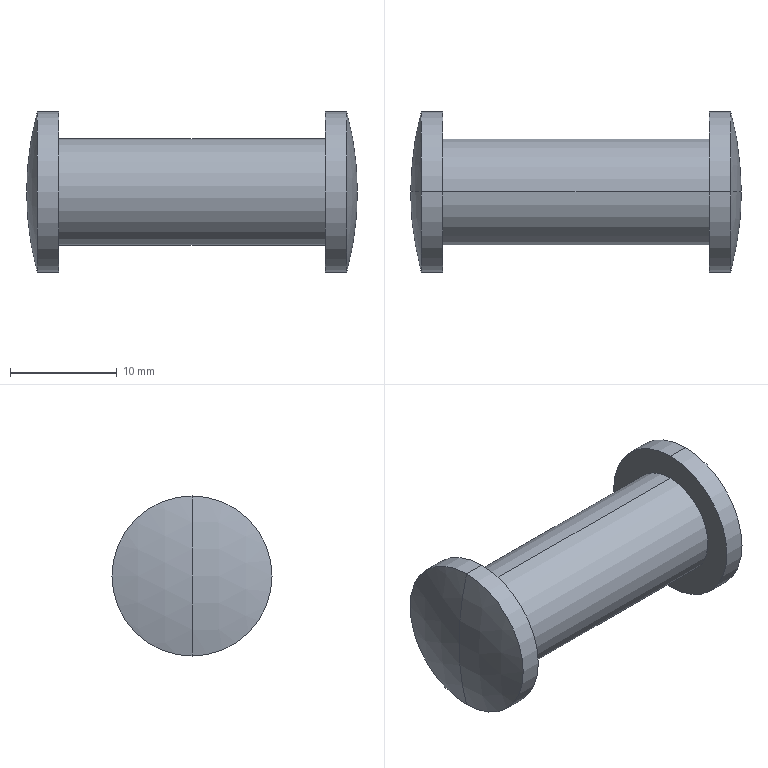Component | SolidWorks | 10x25DowelPin-1 | 1 solid | 12 faces | box 31 x 15 x 15 mm | volume 2848 mm3 | cylinder 6 | sphere 4 | plane 2 | commonest cylinder face diameters 15 x4 10 x2
build123d program:
from build123d import *

# Parameters (mm, degrees)
SKETCH1_R           = 5
BOSS_EXTRUDE1_DEPTH = 12.5
SKETCH2_R           = 7.5
BOSS_EXTRUDE2_DEPTH = 2
DOME1_FACE_RADIUS   = 7.5
DOME1_HEIGHT        = 1
DOME2_FACE_RADIUS   = 7.5
DOME2_HEIGHT        = 1


with BuildPart() as part:
    # Sketch1 → Boss-Extrude1 (new, symmetric)
    with BuildSketch(Plane.XY):
        Circle(SKETCH1_R)
    extrude(amount=BOSS_EXTRUDE1_DEPTH, both=True)

    # Sketch2 → Boss-Extrude2 (add)
    with BuildSketch(Plane.XY.offset(12.5)):
        Circle(SKETCH2_R)
    boss_extrude2 = extrude(amount=BOSS_EXTRUDE2_DEPTH)

    # Mirror1: Boss-Extrude2 across plane
    add(boss_extrude2.mirror(Plane.XY))

    # Dome1: a dome of height H over a round flat face of radius A is a cap of a sphere of radius (A * A + H * H) / (2 * H)
    dome1_r = (DOME1_FACE_RADIUS * DOME1_FACE_RADIUS + DOME1_HEIGHT * DOME1_HEIGHT) / (2 * DOME1_HEIGHT)
    dome1_base = Plane((0, 0, 14.5), z_dir=(0, 0, 1))
    with Locations(dome1_base.offset(DOME1_HEIGHT - dome1_r)):
        dome1_ball = Sphere(dome1_r, mode=Mode.PRIVATE)
    add(split(dome1_ball, bisect_by=dome1_base, keep=Keep.TOP, mode=Mode.PRIVATE))

    # Dome2: a dome of height H over a round flat face of radius A is a cap of a sphere of radius (A * A + H * H) / (2 * H)
    dome2_r = (DOME2_FACE_RADIUS * DOME2_FACE_RADIUS + DOME2_HEIGHT * DOME2_HEIGHT) / (2 * DOME2_HEIGHT)
    dome2_base = Plane((0, 0, -14.5), z_dir=(0, 0, -1))
    with Locations(dome2_base.offset(DOME2_HEIGHT - dome2_r)):
        dome2_ball = Sphere(dome2_r, mode=Mode.PRIVATE)
    add(split(dome2_ball, bisect_by=dome2_base, keep=Keep.TOP, mode=Mode.PRIVATE))


solid = part.part

# Placed as in the assembly
solid = solid.moved(Location((0, -60.308, -258.214), (0, 90, 0)))
STEP:
#1=COLOUR_RGB('',0.7922,0.8196,0.9333);
#2=FILL_AREA_STYLE_COLOUR('',#1);
#3=FILL_AREA_STYLE('',(#2));
#4=SURFACE_STYLE_FILL_AREA(#3);
#5=SURFACE_SIDE_STYLE('',(#4));
#6=SURFACE_STYLE_USAGE(.BOTH.,#5);
#7=PRESENTATION_STYLE_ASSIGNMENT((#6));
#8=CARTESIAN_POINT('',(0.6102,-2.374,-10.166));
#9=VERTEX_POINT('',#8);
#10=CARTESIAN_POINT('',(0.5709,-2.374,-9.871));
#11=VERTEX_POINT('',#10);
#12=CARTESIAN_POINT('',(-0.5167,-2.374,-10.166));
#13=DIRECTION('',(0.,-1.,0.));
#14=DIRECTION('',(0.,0.,-1.));
#15=AXIS2_PLACEMENT_3D('',#12,#13,#14);
#16=CIRCLE('',#15,1.127);
#17=EDGE_CURVE('',#9,#11,#16,.T.);
#18=ORIENTED_EDGE('',*,*,#17,.F.);
#19=CARTESIAN_POINT('',(0.5709,-2.374,-10.461));
#20=VERTEX_POINT('',#19);
#21=CARTESIAN_POINT('',(-0.5167,-2.374,-10.166));
#22=DIRECTION('',(0.,1.,0.));
#23=DIRECTION('',(0.,-0.,1.));
#24=AXIS2_PLACEMENT_3D('',#21,#22,#23);
#25=CIRCLE('',#24,1.127);
#26=EDGE_CURVE('',#9,#20,#25,.T.);
#27=ORIENTED_EDGE('',*,*,#26,.T.);
#28=CARTESIAN_POINT('',(0.5709,-2.374,-10.166));
#29=DIRECTION('',(-1.,0.,0.));
#30=DIRECTION('',(0.,0.,1.));
#31=AXIS2_PLACEMENT_3D('',#28,#29,#30);
#32=CIRCLE('',#31,0.2953);
#33=EDGE_CURVE('',#11,#20,#32,.T.);
#34=ORIENTED_EDGE('',*,*,#33,.F.);
#35=EDGE_LOOP('',(#18,#27,#34));
#36=FACE_OUTER_BOUND('',#35,.T.);
#37=CARTESIAN_POINT('',(-0.5167,-2.374,-10.166));
#38=DIRECTION('',(0.,1.,0.));
#39=DIRECTION('',(0.,0.,1.));
#40=AXIS2_PLACEMENT_3D('',#37,#38,#39);
#41=SPHERICAL_SURFACE('',#40,1.127);
#42=ADVANCED_FACE('',(#36),#41,.T.);
#43=ORIENTED_EDGE('',*,*,#33,.T.);
#44=CARTESIAN_POINT('',(0.4921,-2.374,-10.461));
#45=VERTEX_POINT('',#44);
#46=CARTESIAN_POINT('',(0.5709,-2.374,-10.461));
#47=DIRECTION('',(-1.,0.,0.));
#48=VECTOR('',#47,39.37);
#49=LINE('',#46,#48);
#50=EDGE_CURVE('',#20,#45,#49,.T.);
#51=ORIENTED_EDGE('',*,*,#50,.T.);
#52=CARTESIAN_POINT('',(0.4921,-2.374,-9.871));
#53=VERTEX_POINT('',#52);
#54=CARTESIAN_POINT('',(0.4921,-2.374,-10.166));
#55=DIRECTION('',(-1.,0.,0.));
#56=DIRECTION('',(0.,0.,1.));
#57=AXIS2_PLACEMENT_3D('',#54,#55,#56);
#58=CIRCLE('',#57,0.2953);
#59=EDGE_CURVE('',#53,#45,#58,.T.);
#60=ORIENTED_EDGE('',*,*,#59,.F.);
#61=CARTESIAN_POINT('',(0.5709,-2.374,-9.871));
#62=DIRECTION('',(-1.,0.,0.));
#63=VECTOR('',#62,39.37);
#64=LINE('',#61,#63);
#65=EDGE_CURVE('',#11,#53,#64,.T.);
#66=ORIENTED_EDGE('',*,*,#65,.F.);
#67=EDGE_LOOP('',(#43,#51,#60,#66));
#68=FACE_OUTER_BOUND('',#67,.T.);
#69=CARTESIAN_POINT('',(0.5709,-2.374,-10.166));
#70=DIRECTION('',(-1.,0.,0.));
#71=DIRECTION('',(0.,0.,1.));
#72=AXIS2_PLACEMENT_3D('',#69,#70,#71);
#73=CYLINDRICAL_SURFACE('',#72,0.2953);
#74=ADVANCED_FACE('',(#68),#73,.T.);
#75=CARTESIAN_POINT('',(-0.5709,-2.374,-9.871));
#76=VERTEX_POINT('',#75);
#77=CARTESIAN_POINT('',(-0.5709,-2.374,-10.461));
#78=VERTEX_POINT('',#77);
#79=CARTESIAN_POINT('',(-0.5709,-2.374,-10.166));
#80=DIRECTION('',(-1.,0.,0.));
#81=DIRECTION('',(0.,0.,1.));
#82=AXIS2_PLACEMENT_3D('',#79,#80,#81);
#83=CIRCLE('',#82,0.2953);
#84=EDGE_CURVE('',#76,#78,#83,.T.);
#85=ORIENTED_EDGE('',*,*,#84,.T.);
#86=CARTESIAN_POINT('',(-0.6102,-2.374,-10.166));
#87=VERTEX_POINT('',#86);
#88=CARTESIAN_POINT('',(0.5167,-2.374,-10.166));
#89=DIRECTION('',(0.,1.,0.));
#90=DIRECTION('',(0.,-0.,1.));
#91=AXIS2_PLACEMENT_3D('',#88,#89,#90);
#92=CIRCLE('',#91,1.127);
#93=EDGE_CURVE('',#78,#87,#92,.T.);
#94=ORIENTED_EDGE('',*,*,#93,.T.);
#95=CARTESIAN_POINT('',(0.5167,-2.374,-10.166));
#96=DIRECTION('',(0.,-1.,0.));
#97=DIRECTION('',(0.,0.,-1.));
#98=AXIS2_PLACEMENT_3D('',#95,#96,#97);
#99=CIRCLE('',#98,1.127);
#100=EDGE_CURVE('',#76,#87,#99,.T.);
#101=ORIENTED_EDGE('',*,*,#100,.F.);
#102=EDGE_LOOP('',(#85,#94,#101));
#103=FACE_OUTER_BOUND('',#102,.T.);
#104=CARTESIAN_POINT('',(0.5167,-2.374,-10.166));
#105=DIRECTION('',(0.,1.,0.));
#106=DIRECTION('',(0.,0.,1.));
#107=AXIS2_PLACEMENT_3D('',#104,#105,#106);
#108=SPHERICAL_SURFACE('',#107,1.127);
#109=ADVANCED_FACE('',(#103),#108,.T.);
#110=ORIENTED_EDGE('',*,*,#84,.F.);
#111=CARTESIAN_POINT('',(-0.4921,-2.374,-9.871));
#112=VERTEX_POINT('',#111);
#113=CARTESIAN_POINT('',(-0.5709,-2.374,-9.871));
#114=DIRECTION('',(1.,0.,0.));
#115=VECTOR('',#114,39.37);
#116=LINE('',#113,#115);
#117=EDGE_CURVE('',#76,#112,#116,.T.);
#118=ORIENTED_EDGE('',*,*,#117,.T.);
#119=CARTESIAN_POINT('',(-0.4921,-2.374,-10.461));
#120=VERTEX_POINT('',#119);
#121=CARTESIAN_POINT('',(-0.4921,-2.374,-10.166));
#122=DIRECTION('',(-1.,0.,0.));
#123=DIRECTION('',(0.,0.,1.));
#124=AXIS2_PLACEMENT_3D('',#121,#122,#123);
#125=CIRCLE('',#124,0.2953);
#126=EDGE_CURVE('',#112,#120,#125,.T.);
#127=ORIENTED_EDGE('',*,*,#126,.T.);
#128=CARTESIAN_POINT('',(-0.5709,-2.374,-10.461));
#129=DIRECTION('',(1.,0.,0.));
#130=VECTOR('',#129,39.37);
#131=LINE('',#128,#130);
#132=EDGE_CURVE('',#78,#120,#131,.T.);
#133=ORIENTED_EDGE('',*,*,#132,.F.);
#134=EDGE_LOOP('',(#110,#118,#127,#133));
#135=FACE_OUTER_BOUND('',#134,.T.);
#136=CARTESIAN_POINT('',(-0.5709,-2.374,-10.166));
#137=DIRECTION('',(1.,0.,0.));
#138=DIRECTION('',(0.,0.,-1.));
#139=AXIS2_PLACEMENT_3D('',#136,#137,#138);
#140=CYLINDRICAL_SURFACE('',#139,0.2953);
#141=ADVANCED_FACE('',(#135),#140,.T.);
#142=CARTESIAN_POINT('',(-0.4921,-2.374,-9.969));
#143=VERTEX_POINT('',#142);
#144=CARTESIAN_POINT('',(-0.4921,-2.374,-10.363));
#145=VERTEX_POINT('',#144);
#146=CARTESIAN_POINT('',(-0.4921,-2.374,-10.166));
#147=DIRECTION('',(-1.,0.,0.));
#148=DIRECTION('',(0.,0.,1.));
#149=AXIS2_PLACEMENT_3D('',#146,#147,#148);
#150=CIRCLE('',#149,0.1969);
#151=EDGE_CURVE('',#143,#145,#150,.T.);
#152=ORIENTED_EDGE('',*,*,#151,.F.);
#153=CARTESIAN_POINT('',(0.4921,-2.374,-9.969));
#154=VERTEX_POINT('',#153);
#155=CARTESIAN_POINT('',(-0.4921,-2.374,-9.969));
#156=DIRECTION('',(1.,0.,0.));
#157=VECTOR('',#156,39.37);
#158=LINE('',#155,#157);
#159=EDGE_CURVE('',#143,#154,#158,.T.);
#160=ORIENTED_EDGE('',*,*,#159,.T.);
#161=CARTESIAN_POINT('',(0.4921,-2.374,-10.363));
#162=VERTEX_POINT('',#161);
#163=CARTESIAN_POINT('',(0.4921,-2.374,-10.166));
#164=DIRECTION('',(1.,0.,0.));
#165=DIRECTION('',(0.,0.,-1.));
#166=AXIS2_PLACEMENT_3D('',#163,#164,#165);
#167=CIRCLE('',#166,0.1969);
#168=EDGE_CURVE('',#162,#154,#167,.T.);
#169=ORIENTED_EDGE('',*,*,#168,.F.);
#170=CARTESIAN_POINT('',(-0.4921,-2.374,-10.363));
#171=DIRECTION('',(1.,0.,0.));
#172=VECTOR('',#171,39.37);
#173=LINE('',#170,#172);
#174=EDGE_CURVE('',#145,#162,#173,.T.);
#175=ORIENTED_EDGE('',*,*,#174,.F.);
#176=EDGE_LOOP('',(#152,#160,#169,#175));
#177=FACE_OUTER_BOUND('',#176,.T.);
#178=CARTESIAN_POINT('',(-0.4921,-2.374,-10.166));
#179=DIRECTION('',(1.,0.,0.));
#180=DIRECTION('',(0.,0.,-1.));
#181=AXIS2_PLACEMENT_3D('',#178,#179,#180);
#182=CYLINDRICAL_SURFACE('',#181,0.1969);
#183=ADVANCED_FACE('',(#177),#182,.T.);
#184=ORIENTED_EDGE('',*,*,#159,.F.);
#185=CARTESIAN_POINT('',(-0.4921,-2.374,-10.166));
#186=DIRECTION('',(-1.,0.,0.));
#187=DIRECTION('',(0.,0.,1.));
#188=AXIS2_PLACEMENT_3D('',#185,#186,#187);
#189=CIRCLE('',#188,0.1969);
#190=EDGE_CURVE('',#145,#143,#189,.T.);
#191=ORIENTED_EDGE('',*,*,#190,.F.);
#192=ORIENTED_EDGE('',*,*,#174,.T.);
#193=CARTESIAN_POINT('',(0.4921,-2.374,-10.166));
#194=DIRECTION('',(1.,0.,0.));
#195=DIRECTION('',(0.,0.,-1.));
#196=AXIS2_PLACEMENT_3D('',#193,#194,#195);
#197=CIRCLE('',#196,0.1969);
#198=EDGE_CURVE('',#154,#162,#197,.T.);
#199=ORIENTED_EDGE('',*,*,#198,.F.);
#200=EDGE_LOOP('',(#184,#191,#192,#199));
#201=FACE_OUTER_BOUND('',#200,.T.);
#202=CARTESIAN_POINT('',(-0.4921,-2.374,-10.166));
#203=DIRECTION('',(1.,0.,0.));
#204=DIRECTION('',(0.,0.,-1.));
#205=AXIS2_PLACEMENT_3D('',#202,#203,#204);
#206=CYLINDRICAL_SURFACE('',#205,0.1969);
#207=ADVANCED_FACE('',(#201),#206,.T.);
#208=CARTESIAN_POINT('',(-0.4921,-2.374,-10.166));
#209=DIRECTION('',(-1.,0.,0.));
#210=DIRECTION('',(0.,0.,1.));
#211=AXIS2_PLACEMENT_3D('',#208,#209,#210);
#212=CIRCLE('',#211,0.2953);
#213=EDGE_CURVE('',#120,#112,#212,.T.);
#214=ORIENTED_EDGE('',*,*,#213,.F.);
#215=ORIENTED_EDGE('',*,*,#126,.F.);
#216=EDGE_LOOP('',(#214,#215));
#217=FACE_OUTER_BOUND('',#216,.T.);
#218=ORIENTED_EDGE('',*,*,#190,.T.);
#219=ORIENTED_EDGE('',*,*,#151,.T.);
#220=EDGE_LOOP('',(#218,#219));
#221=FACE_BOUND('',#220,.T.);
#222=CARTESIAN_POINT('',(-0.4921,-2.374,-10.166));
#223=DIRECTION('',(-1.,0.,0.));
#224=DIRECTION('',(0.,0.,1.));
#225=AXIS2_PLACEMENT_3D('',#222,#223,#224);
#226=PLANE('',#225);
#227=ADVANCED_FACE('',(#217,#221),#226,.F.);
#228=ORIENTED_EDGE('',*,*,#117,.F.);
#229=CARTESIAN_POINT('',(-0.5709,-2.374,-10.166));
#230=DIRECTION('',(-1.,0.,0.));
#231=DIRECTION('',(0.,0.,1.));
#232=AXIS2_PLACEMENT_3D('',#229,#230,#231);
#233=CIRCLE('',#232,0.2953);
#234=EDGE_CURVE('',#78,#76,#233,.T.);
#235=ORIENTED_EDGE('',*,*,#234,.F.);
#236=ORIENTED_EDGE('',*,*,#132,.T.);
#237=ORIENTED_EDGE('',*,*,#213,.T.);
#238=EDGE_LOOP('',(#228,#235,#236,#237));
#239=FACE_OUTER_BOUND('',#238,.T.);
#240=CARTESIAN_POINT('',(-0.5709,-2.374,-10.166));
#241=DIRECTION('',(1.,0.,0.));
#242=DIRECTION('',(0.,0.,-1.));
#243=AXIS2_PLACEMENT_3D('',#240,#241,#242);
#244=CYLINDRICAL_SURFACE('',#243,0.2953);
#245=ADVANCED_FACE('',(#239),#244,.T.);
#246=ORIENTED_EDGE('',*,*,#93,.F.);
#247=ORIENTED_EDGE('',*,*,#234,.T.);
#248=ORIENTED_EDGE('',*,*,#100,.T.);
#249=EDGE_LOOP('',(#246,#247,#248));
#250=FACE_OUTER_BOUND('',#249,.T.);
#251=CARTESIAN_POINT('',(0.5167,-2.374,-10.166));
#252=DIRECTION('',(0.,1.,0.));
#253=DIRECTION('',(0.,0.,1.));
#254=AXIS2_PLACEMENT_3D('',#251,#252,#253);
#255=SPHERICAL_SURFACE('',#254,1.127);
#256=ADVANCED_FACE('',(#250),#255,.T.);
#257=ORIENTED_EDGE('',*,*,#59,.T.);
#258=CARTESIAN_POINT('',(0.4921,-2.374,-10.166));
#259=DIRECTION('',(-1.,0.,0.));
#260=DIRECTION('',(0.,0.,1.));
#261=AXIS2_PLACEMENT_3D('',#258,#259,#260);
#262=CIRCLE('',#261,0.2953);
#263=EDGE_CURVE('',#45,#53,#262,.T.);
#264=ORIENTED_EDGE('',*,*,#263,.T.);
#265=EDGE_LOOP('',(#257,#264));
#266=FACE_OUTER_BOUND('',#265,.T.);
#267=ORIENTED_EDGE('',*,*,#168,.T.);
#268=ORIENTED_EDGE('',*,*,#198,.T.);
#269=EDGE_LOOP('',(#267,#268));
#270=FACE_BOUND('',#269,.T.);
#271=CARTESIAN_POINT('',(0.4921,-2.374,-10.166));
#272=DIRECTION('',(1.,0.,0.));
#273=DIRECTION('',(0.,0.,1.));
#274=AXIS2_PLACEMENT_3D('',#271,#272,#273);
#275=PLANE('',#274);
#276=ADVANCED_FACE('',(#266,#270),#275,.F.);
#277=ORIENTED_EDGE('',*,*,#50,.F.);
#278=CARTESIAN_POINT('',(0.5709,-2.374,-10.166));
#279=DIRECTION('',(-1.,0.,0.));
#280=DIRECTION('',(0.,0.,1.));
#281=AXIS2_PLACEMENT_3D('',#278,#279,#280);
#282=CIRCLE('',#281,0.2953);
#283=EDGE_CURVE('',#20,#11,#282,.T.);
#284=ORIENTED_EDGE('',*,*,#283,.T.);
#285=ORIENTED_EDGE('',*,*,#65,.T.);
#286=ORIENTED_EDGE('',*,*,#263,.F.);
#287=EDGE_LOOP('',(#277,#284,#285,#286));
#288=FACE_OUTER_BOUND('',#287,.T.);
#289=CARTESIAN_POINT('',(0.5709,-2.374,-10.166));
#290=DIRECTION('',(-1.,0.,0.));
#291=DIRECTION('',(0.,0.,1.));
#292=AXIS2_PLACEMENT_3D('',#289,#290,#291);
#293=CYLINDRICAL_SURFACE('',#292,0.2953);
#294=ADVANCED_FACE('',(#288),#293,.T.);
#295=ORIENTED_EDGE('',*,*,#26,.F.);
#296=ORIENTED_EDGE('',*,*,#17,.T.);
#297=ORIENTED_EDGE('',*,*,#283,.F.);
#298=EDGE_LOOP('',(#295,#296,#297));
#299=FACE_OUTER_BOUND('',#298,.T.);
#300=CARTESIAN_POINT('',(-0.5167,-2.374,-10.166));
#301=DIRECTION('',(0.,1.,0.));
#302=DIRECTION('',(0.,0.,1.));
#303=AXIS2_PLACEMENT_3D('',#300,#301,#302);
#304=SPHERICAL_SURFACE('',#303,1.127);
#305=ADVANCED_FACE('',(#299),#304,.T.);
#306=CLOSED_SHELL('',(#42,#74,#109,#141,#183,#207,#227,#245,#256,#276,#294,#305));
#307=MANIFOLD_SOLID_BREP('',#306);
#308=STYLED_ITEM('',(#7),#307);
#309=PRESENTATION_LAYER_ASSIGNMENT('','',(#308));
#310=CARTESIAN_POINT('',(0.,0.,0.));
#311=DIRECTION('',(0.,0.,1.));
#312=DIRECTION('',(1.,0.,0.));
#313=AXIS2_PLACEMENT_3D('',#310,#311,#312);
#314=(LENGTH_UNIT()NAMED_UNIT(*)SI_UNIT($,.METRE.));
#315=LENGTH_MEASURE_WITH_UNIT(LENGTH_MEASURE(0.0254),#314);
#316=DIMENSIONAL_EXPONENTS(1.,0.,0.,0.,0.,0.,0.);
#317=(CONVERSION_BASED_UNIT('',#315)LENGTH_UNIT()NAMED_UNIT(#316));
#318=UNCERTAINTY_MEASURE_WITH_UNIT(LENGTH_MEASURE(0.00001),#317,'','');
#319=(NAMED_UNIT(*)PLANE_ANGLE_UNIT()SI_UNIT($,.RADIAN.));
#320=(NAMED_UNIT(*)SI_UNIT($,.STERADIAN.)SOLID_ANGLE_UNIT());
#321=(GEOMETRIC_REPRESENTATION_CONTEXT(3)GLOBAL_UNCERTAINTY_ASSIGNED_CONTEXT((#318))GLOBAL_UNIT_ASSIGNED_CONTEXT((#317,#319,#320))REPRESENTATION_CONTEXT('',''));
#322=ADVANCED_BREP_SHAPE_REPRESENTATION('',(#307,#313),#321);
#323=(LENGTH_UNIT()NAMED_UNIT(*)SI_UNIT($,.METRE.));
#324=LENGTH_MEASURE_WITH_UNIT(LENGTH_MEASURE(0.0254),#323);
#325=DIMENSIONAL_EXPONENTS(1.,0.,0.,0.,0.,0.,0.);
#326=(CONVERSION_BASED_UNIT('',#324)LENGTH_UNIT()NAMED_UNIT(#325));
#327=UNCERTAINTY_MEASURE_WITH_UNIT(LENGTH_MEASURE(0.00001),#326,'','');
#328=(NAMED_UNIT(*)PLANE_ANGLE_UNIT()SI_UNIT($,.RADIAN.));
#329=(NAMED_UNIT(*)SI_UNIT($,.STERADIAN.)SOLID_ANGLE_UNIT());
#330=(GEOMETRIC_REPRESENTATION_CONTEXT(3)GLOBAL_UNCERTAINTY_ASSIGNED_CONTEXT((#327))GLOBAL_UNIT_ASSIGNED_CONTEXT((#326,#328,#329))REPRESENTATION_CONTEXT('',''));
#331=MECHANICAL_DESIGN_GEOMETRIC_PRESENTATION_REPRESENTATION('',(#308),#330);